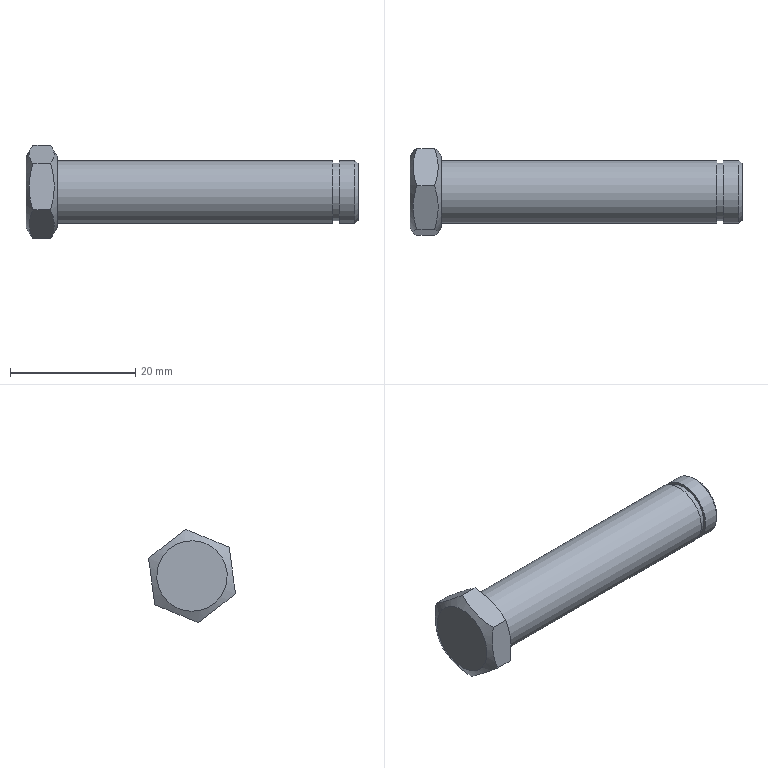Component | NX | ROTATING_SHAFT | 1 solid | 17 faces | volume 4450 mm3 | plane 11 | cylinder 3 | cone 3 | commonest cylinder face diameters 10 x2 9.2 x1